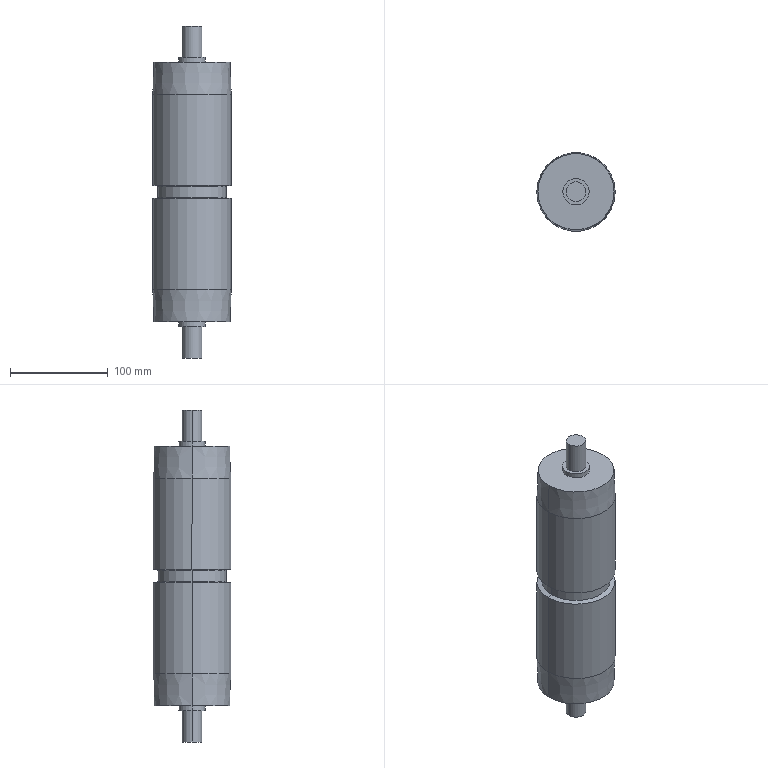Component | SolidWorks | Q1-A12-S21-Q1C.SLDASQ-1_Q1-A12-S21-Q1C-02A-1 | 1 solid | 28 faces | box 80 x 80 x 339.1 mm | volume 1333464 mm3 | cylinder 14 | cone 8 | plane 6 | commonest cylinder face diameters 27 x4 20 x4 80 x4 70 x2 | material SUJ2
build123d program:
from build123d import *


with BuildPart() as part:
    # Sketch1 → Revolve1 (revolve)
    with BuildSketch(Plane.XY, mode=Mode.PRIVATE) as revolve1_sk:
        Polygon((-132.5, 40), (132.5, 40), (132.5, 13.5), (137.45, 13.5), (137.45, 10), (169.55, 10), (169.55, 0), (-169.55, 0), (-169.55, 10), (-137.45, 10), (-137.45, 13.5), (-132.5, 13.5), align=None)
    revolve(revolve1_sk.sketch.rotate(Axis((-250, 0, 0), (1, 0, 0)), 180), axis=Axis((-250, 0, 0), (1, 0, 0)))

    # Sketch4 → Cut-Revolve1 (revolve, cut)
    with BuildSketch(Plane.XY):
        Polygon((-7, 40), (-5.9, 35), (5.9, 35), (7, 40), align=None)
    revolve(axis=Axis((-250, 0, 0), (-1, 0, 0)), mode=Mode.SUBTRACT)

    # Sketch5 → Cut-Revolve2 (revolve, cut)
    with BuildSketch(Plane.XY):
        Polygon((-132.5, 38.865), (-100, 40), (-132.5, 40), align=None)
        Polygon((132.5, 40), (100, 40), (132.5, 38.865), align=None)
    revolve(axis=Axis((-250, 0, 0), (-1, 0, 0)), mode=Mode.SUBTRACT)


solid = part.part

# Placed as in the assembly
solid = solid.moved(Location((2148, 0, 0), (0, 90, 0)))
STEP:
#1=COLOUR_RGB('',0.7922,0.8196,0.9333);
#2=FILL_AREA_STYLE_COLOUR('',#1);
#3=FILL_AREA_STYLE('',(#2));
#4=SURFACE_STYLE_FILL_AREA(#3);
#5=SURFACE_SIDE_STYLE('',(#4));
#6=SURFACE_STYLE_USAGE(.BOTH.,#5);
#7=PRESENTATION_STYLE_ASSIGNMENT((#6));
#8=CARTESIAN_POINT('',(84.035,0.,5.411));
#9=VERTEX_POINT('',#8);
#10=CARTESIAN_POINT('',(85.098,0.,5.411));
#11=VERTEX_POINT('',#10);
#12=CARTESIAN_POINT('',(84.567,0.,5.411));
#13=DIRECTION('',(-0.,-0.,-1.));
#14=DIRECTION('',(-1.,0.,0.));
#15=AXIS2_PLACEMENT_3D('',#12,#13,#14);
#16=CIRCLE('',#15,0.5315);
#17=EDGE_CURVE('',#9,#11,#16,.T.);
#18=ORIENTED_EDGE('',*,*,#17,.T.);
#19=CARTESIAN_POINT('',(85.098,0.,5.217));
#20=VERTEX_POINT('',#19);
#21=CARTESIAN_POINT('',(85.098,0.,-9.843));
#22=DIRECTION('',(-0.,-0.,-1.));
#23=VECTOR('',#22,39.37);
#24=LINE('',#21,#23);
#25=EDGE_CURVE('',#11,#20,#24,.T.);
#26=ORIENTED_EDGE('',*,*,#25,.T.);
#27=CARTESIAN_POINT('',(84.035,0.,5.217));
#28=VERTEX_POINT('',#27);
#29=CARTESIAN_POINT('',(84.567,0.,5.217));
#30=DIRECTION('',(-0.,-0.,-1.));
#31=DIRECTION('',(-1.,0.,0.));
#32=AXIS2_PLACEMENT_3D('',#29,#30,#31);
#33=CIRCLE('',#32,0.5315);
#34=EDGE_CURVE('',#28,#20,#33,.T.);
#35=ORIENTED_EDGE('',*,*,#34,.F.);
#36=CARTESIAN_POINT('',(84.035,0.,-9.843));
#37=DIRECTION('',(-0.,-0.,-1.));
#38=VECTOR('',#37,39.37);
#39=LINE('',#36,#38);
#40=EDGE_CURVE('',#9,#28,#39,.T.);
#41=ORIENTED_EDGE('',*,*,#40,.F.);
#42=EDGE_LOOP('',(#18,#26,#35,#41));
#43=FACE_OUTER_BOUND('',#42,.T.);
#44=CARTESIAN_POINT('',(84.567,0.,-9.843));
#45=DIRECTION('',(-0.,-0.,-1.));
#46=DIRECTION('',(-1.,0.,0.));
#47=AXIS2_PLACEMENT_3D('',#44,#45,#46);
#48=CYLINDRICAL_SURFACE('',#47,0.5315);
#49=ADVANCED_FACE('',(#43),#48,.T.);
#50=CARTESIAN_POINT('',(84.173,0.,6.675));
#51=VERTEX_POINT('',#50);
#52=CARTESIAN_POINT('',(84.961,0.,6.675));
#53=VERTEX_POINT('',#52);
#54=CARTESIAN_POINT('',(84.567,0.,6.675));
#55=DIRECTION('',(-0.,-0.,-1.));
#56=DIRECTION('',(-1.,0.,0.));
#57=AXIS2_PLACEMENT_3D('',#54,#55,#56);
#58=CIRCLE('',#57,0.3937);
#59=EDGE_CURVE('',#51,#53,#58,.T.);
#60=ORIENTED_EDGE('',*,*,#59,.T.);
#61=CARTESIAN_POINT('',(84.961,0.,5.411));
#62=VERTEX_POINT('',#61);
#63=CARTESIAN_POINT('',(84.961,0.,-9.843));
#64=DIRECTION('',(-0.,-0.,-1.));
#65=VECTOR('',#64,39.37);
#66=LINE('',#63,#65);
#67=EDGE_CURVE('',#53,#62,#66,.T.);
#68=ORIENTED_EDGE('',*,*,#67,.T.);
#69=CARTESIAN_POINT('',(84.173,0.,5.411));
#70=VERTEX_POINT('',#69);
#71=CARTESIAN_POINT('',(84.567,0.,5.411));
#72=DIRECTION('',(-0.,-0.,-1.));
#73=DIRECTION('',(-1.,0.,0.));
#74=AXIS2_PLACEMENT_3D('',#71,#72,#73);
#75=CIRCLE('',#74,0.3937);
#76=EDGE_CURVE('',#70,#62,#75,.T.);
#77=ORIENTED_EDGE('',*,*,#76,.F.);
#78=CARTESIAN_POINT('',(84.173,0.,-9.843));
#79=DIRECTION('',(-0.,-0.,-1.));
#80=VECTOR('',#79,39.37);
#81=LINE('',#78,#80);
#82=EDGE_CURVE('',#51,#70,#81,.T.);
#83=ORIENTED_EDGE('',*,*,#82,.F.);
#84=EDGE_LOOP('',(#60,#68,#77,#83));
#85=FACE_OUTER_BOUND('',#84,.T.);
#86=CARTESIAN_POINT('',(84.567,0.,-9.843));
#87=DIRECTION('',(-0.,-0.,-1.));
#88=DIRECTION('',(-1.,0.,0.));
#89=AXIS2_PLACEMENT_3D('',#86,#87,#88);
#90=CYLINDRICAL_SURFACE('',#89,0.3937);
#91=ADVANCED_FACE('',(#85),#90,.T.);
#92=CARTESIAN_POINT('',(86.097,0.,5.217));
#93=VERTEX_POINT('',#92);
#94=CARTESIAN_POINT('',(83.037,0.,5.217));
#95=VERTEX_POINT('',#94);
#96=CARTESIAN_POINT('',(84.567,0.,5.217));
#97=DIRECTION('',(0.,0.,1.));
#98=DIRECTION('',(1.,-0.,0.));
#99=AXIS2_PLACEMENT_3D('',#96,#97,#98);
#100=CIRCLE('',#99,1.53);
#101=EDGE_CURVE('',#93,#95,#100,.T.);
#102=ORIENTED_EDGE('',*,*,#101,.F.);
#103=CARTESIAN_POINT('',(86.142,0.,3.937));
#104=VERTEX_POINT('',#103);
#105=CARTESIAN_POINT('',(86.142,0.,3.937));
#106=DIRECTION('',(0.0349,-0.,-0.9994));
#107=VECTOR('',#106,39.37);
#108=LINE('',#105,#107);
#109=EDGE_CURVE('',#93,#104,#108,.T.);
#110=ORIENTED_EDGE('',*,*,#109,.T.);
#111=CARTESIAN_POINT('',(82.992,0.,3.937));
#112=VERTEX_POINT('',#111);
#113=CARTESIAN_POINT('',(84.567,0.,3.937));
#114=DIRECTION('',(0.,0.,1.));
#115=DIRECTION('',(1.,-0.,0.));
#116=AXIS2_PLACEMENT_3D('',#113,#114,#115);
#117=CIRCLE('',#116,1.575);
#118=EDGE_CURVE('',#104,#112,#117,.T.);
#119=ORIENTED_EDGE('',*,*,#118,.T.);
#120=CARTESIAN_POINT('',(82.992,0.,3.937));
#121=DIRECTION('',(-0.0349,-0.,-0.9994));
#122=VECTOR('',#121,39.37);
#123=LINE('',#120,#122);
#124=EDGE_CURVE('',#95,#112,#123,.T.);
#125=ORIENTED_EDGE('',*,*,#124,.F.);
#126=EDGE_LOOP('',(#102,#110,#119,#125));
#127=FACE_OUTER_BOUND('',#126,.T.);
#128=CARTESIAN_POINT('',(84.567,0.,3.937));
#129=DIRECTION('',(-0.,-0.,-1.));
#130=DIRECTION('',(-1.,0.,0.));
#131=AXIS2_PLACEMENT_3D('',#128,#129,#130);
#132=CONICAL_SURFACE('',#131,1.575,0.03491);
#133=ADVANCED_FACE('',(#127),#132,.T.);
#134=CARTESIAN_POINT('',(84.035,0.,-5.217));
#135=VERTEX_POINT('',#134);
#136=CARTESIAN_POINT('',(85.098,0.,-5.217));
#137=VERTEX_POINT('',#136);
#138=CARTESIAN_POINT('',(84.567,0.,-5.217));
#139=DIRECTION('',(-0.,-0.,-1.));
#140=DIRECTION('',(-1.,0.,0.));
#141=AXIS2_PLACEMENT_3D('',#138,#139,#140);
#142=CIRCLE('',#141,0.5315);
#143=EDGE_CURVE('',#135,#137,#142,.T.);
#144=ORIENTED_EDGE('',*,*,#143,.T.);
#145=CARTESIAN_POINT('',(85.098,0.,-5.411));
#146=VERTEX_POINT('',#145);
#147=CARTESIAN_POINT('',(85.098,0.,-9.843));
#148=DIRECTION('',(-0.,-0.,-1.));
#149=VECTOR('',#148,39.37);
#150=LINE('',#147,#149);
#151=EDGE_CURVE('',#137,#146,#150,.T.);
#152=ORIENTED_EDGE('',*,*,#151,.T.);
#153=CARTESIAN_POINT('',(84.035,0.,-5.411));
#154=VERTEX_POINT('',#153);
#155=CARTESIAN_POINT('',(84.567,0.,-5.411));
#156=DIRECTION('',(-0.,-0.,-1.));
#157=DIRECTION('',(-1.,0.,0.));
#158=AXIS2_PLACEMENT_3D('',#155,#156,#157);
#159=CIRCLE('',#158,0.5315);
#160=EDGE_CURVE('',#154,#146,#159,.T.);
#161=ORIENTED_EDGE('',*,*,#160,.F.);
#162=CARTESIAN_POINT('',(84.035,0.,-9.843));
#163=DIRECTION('',(-0.,-0.,-1.));
#164=VECTOR('',#163,39.37);
#165=LINE('',#162,#164);
#166=EDGE_CURVE('',#135,#154,#165,.T.);
#167=ORIENTED_EDGE('',*,*,#166,.F.);
#168=EDGE_LOOP('',(#144,#152,#161,#167));
#169=FACE_OUTER_BOUND('',#168,.T.);
#170=CARTESIAN_POINT('',(84.567,0.,-9.843));
#171=DIRECTION('',(-0.,-0.,-1.));
#172=DIRECTION('',(-1.,0.,0.));
#173=AXIS2_PLACEMENT_3D('',#170,#171,#172);
#174=CYLINDRICAL_SURFACE('',#173,0.5315);
#175=ADVANCED_FACE('',(#169),#174,.T.);
#176=CARTESIAN_POINT('',(84.173,0.,-5.411));
#177=VERTEX_POINT('',#176);
#178=CARTESIAN_POINT('',(84.961,0.,-5.411));
#179=VERTEX_POINT('',#178);
#180=CARTESIAN_POINT('',(84.567,0.,-5.411));
#181=DIRECTION('',(-0.,-0.,-1.));
#182=DIRECTION('',(-1.,0.,0.));
#183=AXIS2_PLACEMENT_3D('',#180,#181,#182);
#184=CIRCLE('',#183,0.3937);
#185=EDGE_CURVE('',#177,#179,#184,.T.);
#186=ORIENTED_EDGE('',*,*,#185,.T.);
#187=CARTESIAN_POINT('',(84.961,0.,-6.675));
#188=VERTEX_POINT('',#187);
#189=CARTESIAN_POINT('',(84.961,0.,-9.843));
#190=DIRECTION('',(-0.,-0.,-1.));
#191=VECTOR('',#190,39.37);
#192=LINE('',#189,#191);
#193=EDGE_CURVE('',#179,#188,#192,.T.);
#194=ORIENTED_EDGE('',*,*,#193,.T.);
#195=CARTESIAN_POINT('',(84.173,0.,-6.675));
#196=VERTEX_POINT('',#195);
#197=CARTESIAN_POINT('',(84.567,0.,-6.675));
#198=DIRECTION('',(-0.,-0.,-1.));
#199=DIRECTION('',(-1.,0.,0.));
#200=AXIS2_PLACEMENT_3D('',#197,#198,#199);
#201=CIRCLE('',#200,0.3937);
#202=EDGE_CURVE('',#196,#188,#201,.T.);
#203=ORIENTED_EDGE('',*,*,#202,.F.);
#204=CARTESIAN_POINT('',(84.173,0.,-9.843));
#205=DIRECTION('',(-0.,-0.,-1.));
#206=VECTOR('',#205,39.37);
#207=LINE('',#204,#206);
#208=EDGE_CURVE('',#177,#196,#207,.T.);
#209=ORIENTED_EDGE('',*,*,#208,.F.);
#210=EDGE_LOOP('',(#186,#194,#203,#209));
#211=FACE_OUTER_BOUND('',#210,.T.);
#212=CARTESIAN_POINT('',(84.567,0.,-9.843));
#213=DIRECTION('',(-0.,-0.,-1.));
#214=DIRECTION('',(-1.,0.,0.));
#215=AXIS2_PLACEMENT_3D('',#212,#213,#214);
#216=CYLINDRICAL_SURFACE('',#215,0.3937);
#217=ADVANCED_FACE('',(#211),#216,.T.);
#218=CARTESIAN_POINT('',(86.097,0.,-5.217));
#219=VERTEX_POINT('',#218);
#220=CARTESIAN_POINT('',(83.037,0.,-5.217));
#221=VERTEX_POINT('',#220);
#222=CARTESIAN_POINT('',(84.567,0.,-5.217));
#223=DIRECTION('',(0.,0.,1.));
#224=DIRECTION('',(1.,-0.,0.));
#225=AXIS2_PLACEMENT_3D('',#222,#223,#224);
#226=CIRCLE('',#225,1.53);
#227=EDGE_CURVE('',#219,#221,#226,.T.);
#228=ORIENTED_EDGE('',*,*,#227,.T.);
#229=CARTESIAN_POINT('',(82.992,0.,-3.937));
#230=VERTEX_POINT('',#229);
#231=CARTESIAN_POINT('',(83.037,0.,-5.217));
#232=DIRECTION('',(-0.0349,0.,0.9994));
#233=VECTOR('',#232,39.37);
#234=LINE('',#231,#233);
#235=EDGE_CURVE('',#221,#230,#234,.T.);
#236=ORIENTED_EDGE('',*,*,#235,.T.);
#237=CARTESIAN_POINT('',(86.142,0.,-3.937));
#238=VERTEX_POINT('',#237);
#239=CARTESIAN_POINT('',(84.567,0.,-3.937));
#240=DIRECTION('',(0.,0.,1.));
#241=DIRECTION('',(1.,-0.,0.));
#242=AXIS2_PLACEMENT_3D('',#239,#240,#241);
#243=CIRCLE('',#242,1.575);
#244=EDGE_CURVE('',#238,#230,#243,.T.);
#245=ORIENTED_EDGE('',*,*,#244,.F.);
#246=CARTESIAN_POINT('',(86.097,0.,-5.217));
#247=DIRECTION('',(0.0349,0.,0.9994));
#248=VECTOR('',#247,39.37);
#249=LINE('',#246,#248);
#250=EDGE_CURVE('',#219,#238,#249,.T.);
#251=ORIENTED_EDGE('',*,*,#250,.F.);
#252=EDGE_LOOP('',(#228,#236,#245,#251));
#253=FACE_OUTER_BOUND('',#252,.T.);
#254=CARTESIAN_POINT('',(84.567,0.,-5.217));
#255=DIRECTION('',(0.,0.,1.));
#256=DIRECTION('',(1.,-0.,0.));
#257=AXIS2_PLACEMENT_3D('',#254,#255,#256);
#258=CONICAL_SURFACE('',#257,1.53,0.03491);
#259=ADVANCED_FACE('',(#253),#258,.T.);
#260=ORIENTED_EDGE('',*,*,#118,.F.);
#261=CARTESIAN_POINT('',(86.142,0.,0.2756));
#262=VERTEX_POINT('',#261);
#263=CARTESIAN_POINT('',(86.142,0.,-9.843));
#264=DIRECTION('',(-0.,-0.,-1.));
#265=VECTOR('',#264,39.37);
#266=LINE('',#263,#265);
#267=EDGE_CURVE('',#104,#262,#266,.T.);
#268=ORIENTED_EDGE('',*,*,#267,.T.);
#269=CARTESIAN_POINT('',(82.992,0.,0.2756));
#270=VERTEX_POINT('',#269);
#271=CARTESIAN_POINT('',(84.567,0.,0.2756));
#272=DIRECTION('',(0.,0.,1.));
#273=DIRECTION('',(1.,-0.,-0.));
#274=AXIS2_PLACEMENT_3D('',#271,#272,#273);
#275=CIRCLE('',#274,1.575);
#276=EDGE_CURVE('',#262,#270,#275,.T.);
#277=ORIENTED_EDGE('',*,*,#276,.T.);
#278=CARTESIAN_POINT('',(82.992,0.,-9.843));
#279=DIRECTION('',(-0.,-0.,-1.));
#280=VECTOR('',#279,39.37);
#281=LINE('',#278,#280);
#282=EDGE_CURVE('',#112,#270,#281,.T.);
#283=ORIENTED_EDGE('',*,*,#282,.F.);
#284=EDGE_LOOP('',(#260,#268,#277,#283));
#285=FACE_OUTER_BOUND('',#284,.T.);
#286=CARTESIAN_POINT('',(84.567,0.,-9.843));
#287=DIRECTION('',(-0.,-0.,-1.));
#288=DIRECTION('',(-1.,0.,0.));
#289=AXIS2_PLACEMENT_3D('',#286,#287,#288);
#290=CYLINDRICAL_SURFACE('',#289,1.575);
#291=ADVANCED_FACE('',(#285),#290,.T.);
#292=CARTESIAN_POINT('',(85.945,0.,0.2323));
#293=VERTEX_POINT('',#292);
#294=CARTESIAN_POINT('',(83.189,0.,0.2323));
#295=VERTEX_POINT('',#294);
#296=CARTESIAN_POINT('',(84.567,0.,0.2323));
#297=DIRECTION('',(0.,0.,1.));
#298=DIRECTION('',(1.,-0.,-0.));
#299=AXIS2_PLACEMENT_3D('',#296,#297,#298);
#300=CIRCLE('',#299,1.378);
#301=EDGE_CURVE('',#293,#295,#300,.T.);
#302=ORIENTED_EDGE('',*,*,#301,.T.);
#303=CARTESIAN_POINT('',(83.189,0.,0.2323));
#304=DIRECTION('',(-0.9766,0.,0.2149));
#305=VECTOR('',#304,39.37);
#306=LINE('',#303,#305);
#307=EDGE_CURVE('',#295,#270,#306,.T.);
#308=ORIENTED_EDGE('',*,*,#307,.T.);
#309=ORIENTED_EDGE('',*,*,#276,.F.);
#310=CARTESIAN_POINT('',(85.945,0.,0.2323));
#311=DIRECTION('',(0.9766,-0.,0.2149));
#312=VECTOR('',#311,39.37);
#313=LINE('',#310,#312);
#314=EDGE_CURVE('',#293,#262,#313,.T.);
#315=ORIENTED_EDGE('',*,*,#314,.F.);
#316=EDGE_LOOP('',(#302,#308,#309,#315));
#317=FACE_OUTER_BOUND('',#316,.T.);
#318=CARTESIAN_POINT('',(84.567,0.,0.2323));
#319=DIRECTION('',(0.,0.,1.));
#320=DIRECTION('',(1.,-0.,-0.));
#321=AXIS2_PLACEMENT_3D('',#318,#319,#320);
#322=CONICAL_SURFACE('',#321,1.378,1.354);
#323=ADVANCED_FACE('',(#317),#322,.T.);
#324=CARTESIAN_POINT('',(85.945,0.,-0.2323));
#325=VERTEX_POINT('',#324);
#326=CARTESIAN_POINT('',(83.189,0.,-0.2323));
#327=VERTEX_POINT('',#326);
#328=CARTESIAN_POINT('',(84.567,0.,-0.2323));
#329=DIRECTION('',(0.,0.,1.));
#330=DIRECTION('',(1.,-0.,-0.));
#331=AXIS2_PLACEMENT_3D('',#328,#329,#330);
#332=CIRCLE('',#331,1.378);
#333=EDGE_CURVE('',#325,#327,#332,.T.);
#334=ORIENTED_EDGE('',*,*,#333,.T.);
#335=CARTESIAN_POINT('',(83.189,0.,5.217));
#336=DIRECTION('',(0.,0.,1.));
#337=VECTOR('',#336,39.37);
#338=LINE('',#335,#337);
#339=EDGE_CURVE('',#327,#295,#338,.T.);
#340=ORIENTED_EDGE('',*,*,#339,.T.);
#341=ORIENTED_EDGE('',*,*,#301,.F.);
#342=CARTESIAN_POINT('',(85.945,0.,5.217));
#343=DIRECTION('',(0.,0.,1.));
#344=VECTOR('',#343,39.37);
#345=LINE('',#342,#344);
#346=EDGE_CURVE('',#325,#293,#345,.T.);
#347=ORIENTED_EDGE('',*,*,#346,.F.);
#348=EDGE_LOOP('',(#334,#340,#341,#347));
#349=FACE_OUTER_BOUND('',#348,.T.);
#350=CARTESIAN_POINT('',(84.567,0.,5.217));
#351=DIRECTION('',(0.,0.,1.));
#352=DIRECTION('',(1.,-0.,0.));
#353=AXIS2_PLACEMENT_3D('',#350,#351,#352);
#354=CYLINDRICAL_SURFACE('',#353,1.378);
#355=ADVANCED_FACE('',(#349),#354,.T.);
#356=ORIENTED_EDGE('',*,*,#333,.F.);
#357=CARTESIAN_POINT('',(86.142,0.,-0.2756));
#358=VERTEX_POINT('',#357);
#359=CARTESIAN_POINT('',(86.142,0.,-0.2756));
#360=DIRECTION('',(0.9766,0.,-0.2149));
#361=VECTOR('',#360,39.37);
#362=LINE('',#359,#361);
#363=EDGE_CURVE('',#325,#358,#362,.T.);
#364=ORIENTED_EDGE('',*,*,#363,.T.);
#365=CARTESIAN_POINT('',(82.992,0.,-0.2756));
#366=VERTEX_POINT('',#365);
#367=CARTESIAN_POINT('',(84.567,0.,-0.2756));
#368=DIRECTION('',(0.,0.,1.));
#369=DIRECTION('',(1.,-0.,-0.));
#370=AXIS2_PLACEMENT_3D('',#367,#368,#369);
#371=CIRCLE('',#370,1.575);
#372=EDGE_CURVE('',#358,#366,#371,.T.);
#373=ORIENTED_EDGE('',*,*,#372,.T.);
#374=CARTESIAN_POINT('',(82.992,0.,-0.2756));
#375=DIRECTION('',(-0.9766,0.,-0.2149));
#376=VECTOR('',#375,39.37);
#377=LINE('',#374,#376);
#378=EDGE_CURVE('',#327,#366,#377,.T.);
#379=ORIENTED_EDGE('',*,*,#378,.F.);
#380=EDGE_LOOP('',(#356,#364,#373,#379));
#381=FACE_OUTER_BOUND('',#380,.T.);
#382=CARTESIAN_POINT('',(84.567,0.,-0.2756));
#383=DIRECTION('',(-0.,-0.,-1.));
#384=DIRECTION('',(-1.,0.,0.));
#385=AXIS2_PLACEMENT_3D('',#382,#383,#384);
#386=CONICAL_SURFACE('',#385,1.575,1.354);
#387=ADVANCED_FACE('',(#381),#386,.T.);
#388=ORIENTED_EDGE('',*,*,#372,.F.);
#389=CARTESIAN_POINT('',(86.142,0.,-9.843));
#390=DIRECTION('',(-0.,-0.,-1.));
#391=VECTOR('',#390,39.37);
#392=LINE('',#389,#391);
#393=EDGE_CURVE('',#358,#238,#392,.T.);
#394=ORIENTED_EDGE('',*,*,#393,.T.);
#395=ORIENTED_EDGE('',*,*,#244,.T.);
#396=CARTESIAN_POINT('',(82.992,0.,-9.843));
#397=DIRECTION('',(-0.,-0.,-1.));
#398=VECTOR('',#397,39.37);
#399=LINE('',#396,#398);
#400=EDGE_CURVE('',#366,#230,#399,.T.);
#401=ORIENTED_EDGE('',*,*,#400,.F.);
#402=EDGE_LOOP('',(#388,#394,#395,#401));
#403=FACE_OUTER_BOUND('',#402,.T.);
#404=CARTESIAN_POINT('',(84.567,0.,-9.843));
#405=DIRECTION('',(-0.,-0.,-1.));
#406=DIRECTION('',(-1.,0.,0.));
#407=AXIS2_PLACEMENT_3D('',#404,#405,#406);
#408=CYLINDRICAL_SURFACE('',#407,1.575);
#409=ADVANCED_FACE('',(#403),#408,.T.);
#410=ORIENTED_EDGE('',*,*,#393,.F.);
#411=CARTESIAN_POINT('',(84.567,0.,-0.2756));
#412=DIRECTION('',(0.,0.,1.));
#413=DIRECTION('',(1.,-0.,-0.));
#414=AXIS2_PLACEMENT_3D('',#411,#412,#413);
#415=CIRCLE('',#414,1.575);
#416=EDGE_CURVE('',#366,#358,#415,.T.);
#417=ORIENTED_EDGE('',*,*,#416,.F.);
#418=ORIENTED_EDGE('',*,*,#400,.T.);
#419=CARTESIAN_POINT('',(84.567,0.,-3.937));
#420=DIRECTION('',(0.,0.,1.));
#421=DIRECTION('',(1.,-0.,0.));
#422=AXIS2_PLACEMENT_3D('',#419,#420,#421);
#423=CIRCLE('',#422,1.575);
#424=EDGE_CURVE('',#230,#238,#423,.T.);
#425=ORIENTED_EDGE('',*,*,#424,.T.);
#426=EDGE_LOOP('',(#410,#417,#418,#425));
#427=FACE_OUTER_BOUND('',#426,.T.);
#428=CARTESIAN_POINT('',(84.567,0.,-9.843));
#429=DIRECTION('',(-0.,-0.,-1.));
#430=DIRECTION('',(-1.,0.,0.));
#431=AXIS2_PLACEMENT_3D('',#428,#429,#430);
#432=CYLINDRICAL_SURFACE('',#431,1.575);
#433=ADVANCED_FACE('',(#427),#432,.T.);
#434=ORIENTED_EDGE('',*,*,#363,.F.);
#435=CARTESIAN_POINT('',(84.567,0.,-0.2323));
#436=DIRECTION('',(0.,0.,1.));
#437=DIRECTION('',(1.,-0.,-0.));
#438=AXIS2_PLACEMENT_3D('',#435,#436,#437);
#439=CIRCLE('',#438,1.378);
#440=EDGE_CURVE('',#327,#325,#439,.T.);
#441=ORIENTED_EDGE('',*,*,#440,.F.);
#442=ORIENTED_EDGE('',*,*,#378,.T.);
#443=ORIENTED_EDGE('',*,*,#416,.T.);
#444=EDGE_LOOP('',(#434,#441,#442,#443));
#445=FACE_OUTER_BOUND('',#444,.T.);
#446=CARTESIAN_POINT('',(84.567,0.,-0.2756));
#447=DIRECTION('',(-0.,-0.,-1.));
#448=DIRECTION('',(-1.,0.,0.));
#449=AXIS2_PLACEMENT_3D('',#446,#447,#448);
#450=CONICAL_SURFACE('',#449,1.575,1.354);
#451=ADVANCED_FACE('',(#445),#450,.T.);
#452=ORIENTED_EDGE('',*,*,#339,.F.);
#453=ORIENTED_EDGE('',*,*,#440,.T.);
#454=ORIENTED_EDGE('',*,*,#346,.T.);
#455=CARTESIAN_POINT('',(84.567,0.,0.2323));
#456=DIRECTION('',(0.,0.,1.));
#457=DIRECTION('',(1.,-0.,-0.));
#458=AXIS2_PLACEMENT_3D('',#455,#456,#457);
#459=CIRCLE('',#458,1.378);
#460=EDGE_CURVE('',#295,#293,#459,.T.);
#461=ORIENTED_EDGE('',*,*,#460,.F.);
#462=EDGE_LOOP('',(#452,#453,#454,#461));
#463=FACE_OUTER_BOUND('',#462,.T.);
#464=CARTESIAN_POINT('',(84.567,0.,5.217));
#465=DIRECTION('',(0.,0.,1.));
#466=DIRECTION('',(1.,-0.,0.));
#467=AXIS2_PLACEMENT_3D('',#464,#465,#466);
#468=CYLINDRICAL_SURFACE('',#467,1.378);
#469=ADVANCED_FACE('',(#463),#468,.T.);
#470=ORIENTED_EDGE('',*,*,#307,.F.);
#471=ORIENTED_EDGE('',*,*,#460,.T.);
#472=ORIENTED_EDGE('',*,*,#314,.T.);
#473=CARTESIAN_POINT('',(84.567,0.,0.2756));
#474=DIRECTION('',(0.,0.,1.));
#475=DIRECTION('',(1.,-0.,-0.));
#476=AXIS2_PLACEMENT_3D('',#473,#474,#475);
#477=CIRCLE('',#476,1.575);
#478=EDGE_CURVE('',#270,#262,#477,.T.);
#479=ORIENTED_EDGE('',*,*,#478,.F.);
#480=EDGE_LOOP('',(#470,#471,#472,#479));
#481=FACE_OUTER_BOUND('',#480,.T.);
#482=CARTESIAN_POINT('',(84.567,0.,0.2323));
#483=DIRECTION('',(0.,0.,1.));
#484=DIRECTION('',(1.,-0.,-0.));
#485=AXIS2_PLACEMENT_3D('',#482,#483,#484);
#486=CONICAL_SURFACE('',#485,1.378,1.354);
#487=ADVANCED_FACE('',(#481),#486,.T.);
#488=ORIENTED_EDGE('',*,*,#267,.F.);
#489=CARTESIAN_POINT('',(84.567,0.,3.937));
#490=DIRECTION('',(0.,0.,1.));
#491=DIRECTION('',(1.,-0.,0.));
#492=AXIS2_PLACEMENT_3D('',#489,#490,#491);
#493=CIRCLE('',#492,1.575);
#494=EDGE_CURVE('',#112,#104,#493,.T.);
#495=ORIENTED_EDGE('',*,*,#494,.F.);
#496=ORIENTED_EDGE('',*,*,#282,.T.);
#497=ORIENTED_EDGE('',*,*,#478,.T.);
#498=EDGE_LOOP('',(#488,#495,#496,#497));
#499=FACE_OUTER_BOUND('',#498,.T.);
#500=CARTESIAN_POINT('',(84.567,0.,-9.843));
#501=DIRECTION('',(-0.,-0.,-1.));
#502=DIRECTION('',(-1.,0.,0.));
#503=AXIS2_PLACEMENT_3D('',#500,#501,#502);
#504=CYLINDRICAL_SURFACE('',#503,1.575);
#505=ADVANCED_FACE('',(#499),#504,.T.);
#506=ORIENTED_EDGE('',*,*,#235,.F.);
#507=CARTESIAN_POINT('',(84.567,0.,-5.217));
#508=DIRECTION('',(0.,0.,1.));
#509=DIRECTION('',(1.,-0.,0.));
#510=AXIS2_PLACEMENT_3D('',#507,#508,#509);
#511=CIRCLE('',#510,1.53);
#512=EDGE_CURVE('',#221,#219,#511,.T.);
#513=ORIENTED_EDGE('',*,*,#512,.T.);
#514=ORIENTED_EDGE('',*,*,#250,.T.);
#515=ORIENTED_EDGE('',*,*,#424,.F.);
#516=EDGE_LOOP('',(#506,#513,#514,#515));
#517=FACE_OUTER_BOUND('',#516,.T.);
#518=CARTESIAN_POINT('',(84.567,0.,-5.217));
#519=DIRECTION('',(0.,0.,1.));
#520=DIRECTION('',(1.,-0.,0.));
#521=AXIS2_PLACEMENT_3D('',#518,#519,#520);
#522=CONICAL_SURFACE('',#521,1.53,0.03491);
#523=ADVANCED_FACE('',(#517),#522,.T.);
#524=ORIENTED_EDGE('',*,*,#202,.T.);
#525=CARTESIAN_POINT('',(84.567,0.,-6.675));
#526=DIRECTION('',(-0.,-0.,-1.));
#527=DIRECTION('',(-1.,0.,0.));
#528=AXIS2_PLACEMENT_3D('',#525,#526,#527);
#529=CIRCLE('',#528,0.3937);
#530=EDGE_CURVE('',#188,#196,#529,.T.);
#531=ORIENTED_EDGE('',*,*,#530,.T.);
#532=EDGE_LOOP('',(#524,#531));
#533=FACE_OUTER_BOUND('',#532,.T.);
#534=CARTESIAN_POINT('',(84.961,0.,-6.675));
#535=DIRECTION('',(0.,0.,1.));
#536=DIRECTION('',(1.,-0.,-0.));
#537=AXIS2_PLACEMENT_3D('',#534,#535,#536);
#538=PLANE('',#537);
#539=ADVANCED_FACE('',(#533),#538,.F.);
#540=ORIENTED_EDGE('',*,*,#193,.F.);
#541=CARTESIAN_POINT('',(84.567,0.,-5.411));
#542=DIRECTION('',(-0.,-0.,-1.));
#543=DIRECTION('',(-1.,0.,0.));
#544=AXIS2_PLACEMENT_3D('',#541,#542,#543);
#545=CIRCLE('',#544,0.3937);
#546=EDGE_CURVE('',#179,#177,#545,.T.);
#547=ORIENTED_EDGE('',*,*,#546,.T.);
#548=ORIENTED_EDGE('',*,*,#208,.T.);
#549=ORIENTED_EDGE('',*,*,#530,.F.);
#550=EDGE_LOOP('',(#540,#547,#548,#549));
#551=FACE_OUTER_BOUND('',#550,.T.);
#552=CARTESIAN_POINT('',(84.567,0.,-9.843));
#553=DIRECTION('',(-0.,-0.,-1.));
#554=DIRECTION('',(-1.,0.,0.));
#555=AXIS2_PLACEMENT_3D('',#552,#553,#554);
#556=CYLINDRICAL_SURFACE('',#555,0.3937);
#557=ADVANCED_FACE('',(#551),#556,.T.);
#558=ORIENTED_EDGE('',*,*,#185,.F.);
#559=ORIENTED_EDGE('',*,*,#546,.F.);
#560=EDGE_LOOP('',(#558,#559));
#561=FACE_BOUND('',#560,.T.);
#562=ORIENTED_EDGE('',*,*,#160,.T.);
#563=CARTESIAN_POINT('',(84.567,0.,-5.411));
#564=DIRECTION('',(-0.,-0.,-1.));
#565=DIRECTION('',(-1.,0.,0.));
#566=AXIS2_PLACEMENT_3D('',#563,#564,#565);
#567=CIRCLE('',#566,0.5315);
#568=EDGE_CURVE('',#146,#154,#567,.T.);
#569=ORIENTED_EDGE('',*,*,#568,.T.);
#570=EDGE_LOOP('',(#562,#569));
#571=FACE_OUTER_BOUND('',#570,.T.);
#572=CARTESIAN_POINT('',(85.098,0.,-5.411));
#573=DIRECTION('',(0.,0.,1.));
#574=DIRECTION('',(1.,-0.,-0.));
#575=AXIS2_PLACEMENT_3D('',#572,#573,#574);
#576=PLANE('',#575);
#577=ADVANCED_FACE('',(#561,#571),#576,.F.);
#578=ORIENTED_EDGE('',*,*,#151,.F.);
#579=CARTESIAN_POINT('',(84.567,0.,-5.217));
#580=DIRECTION('',(-0.,-0.,-1.));
#581=DIRECTION('',(-1.,0.,0.));
#582=AXIS2_PLACEMENT_3D('',#579,#580,#581);
#583=CIRCLE('',#582,0.5315);
#584=EDGE_CURVE('',#137,#135,#583,.T.);
#585=ORIENTED_EDGE('',*,*,#584,.T.);
#586=ORIENTED_EDGE('',*,*,#166,.T.);
#587=ORIENTED_EDGE('',*,*,#568,.F.);
#588=EDGE_LOOP('',(#578,#585,#586,#587));
#589=FACE_OUTER_BOUND('',#588,.T.);
#590=CARTESIAN_POINT('',(84.567,0.,-9.843));
#591=DIRECTION('',(-0.,-0.,-1.));
#592=DIRECTION('',(-1.,0.,0.));
#593=AXIS2_PLACEMENT_3D('',#590,#591,#592);
#594=CYLINDRICAL_SURFACE('',#593,0.5315);
#595=ADVANCED_FACE('',(#589),#594,.T.);
#596=ORIENTED_EDGE('',*,*,#143,.F.);
#597=ORIENTED_EDGE('',*,*,#584,.F.);
#598=EDGE_LOOP('',(#596,#597));
#599=FACE_BOUND('',#598,.T.);
#600=ORIENTED_EDGE('',*,*,#227,.F.);
#601=ORIENTED_EDGE('',*,*,#512,.F.);
#602=EDGE_LOOP('',(#600,#601));
#603=FACE_OUTER_BOUND('',#602,.T.);
#604=CARTESIAN_POINT('',(85.098,0.,-5.217));
#605=DIRECTION('',(0.,0.,1.));
#606=DIRECTION('',(1.,-0.,-0.));
#607=AXIS2_PLACEMENT_3D('',#604,#605,#606);
#608=PLANE('',#607);
#609=ADVANCED_FACE('',(#599,#603),#608,.F.);
#610=ORIENTED_EDGE('',*,*,#109,.F.);
#611=CARTESIAN_POINT('',(84.567,0.,5.217));
#612=DIRECTION('',(0.,0.,1.));
#613=DIRECTION('',(1.,-0.,0.));
#614=AXIS2_PLACEMENT_3D('',#611,#612,#613);
#615=CIRCLE('',#614,1.53);
#616=EDGE_CURVE('',#95,#93,#615,.T.);
#617=ORIENTED_EDGE('',*,*,#616,.F.);
#618=ORIENTED_EDGE('',*,*,#124,.T.);
#619=ORIENTED_EDGE('',*,*,#494,.T.);
#620=EDGE_LOOP('',(#610,#617,#618,#619));
#621=FACE_OUTER_BOUND('',#620,.T.);
#622=CARTESIAN_POINT('',(84.567,0.,3.937));
#623=DIRECTION('',(-0.,-0.,-1.));
#624=DIRECTION('',(-1.,0.,0.));
#625=AXIS2_PLACEMENT_3D('',#622,#623,#624);
#626=CONICAL_SURFACE('',#625,1.575,0.03491);
#627=ADVANCED_FACE('',(#621),#626,.T.);
#628=ORIENTED_EDGE('',*,*,#59,.F.);
#629=CARTESIAN_POINT('',(84.567,0.,6.675));
#630=DIRECTION('',(-0.,-0.,-1.));
#631=DIRECTION('',(-1.,0.,0.));
#632=AXIS2_PLACEMENT_3D('',#629,#630,#631);
#633=CIRCLE('',#632,0.3937);
#634=EDGE_CURVE('',#53,#51,#633,.T.);
#635=ORIENTED_EDGE('',*,*,#634,.F.);
#636=EDGE_LOOP('',(#628,#635));
#637=FACE_OUTER_BOUND('',#636,.T.);
#638=CARTESIAN_POINT('',(84.961,0.,6.675));
#639=DIRECTION('',(-0.,-0.,-1.));
#640=DIRECTION('',(-1.,0.,0.));
#641=AXIS2_PLACEMENT_3D('',#638,#639,#640);
#642=PLANE('',#641);
#643=ADVANCED_FACE('',(#637),#642,.F.);
#644=ORIENTED_EDGE('',*,*,#67,.F.);
#645=ORIENTED_EDGE('',*,*,#634,.T.);
#646=ORIENTED_EDGE('',*,*,#82,.T.);
#647=CARTESIAN_POINT('',(84.567,0.,5.411));
#648=DIRECTION('',(-0.,-0.,-1.));
#649=DIRECTION('',(-1.,0.,0.));
#650=AXIS2_PLACEMENT_3D('',#647,#648,#649);
#651=CIRCLE('',#650,0.3937);
#652=EDGE_CURVE('',#62,#70,#651,.T.);
#653=ORIENTED_EDGE('',*,*,#652,.F.);
#654=EDGE_LOOP('',(#644,#645,#646,#653));
#655=FACE_OUTER_BOUND('',#654,.T.);
#656=CARTESIAN_POINT('',(84.567,0.,-9.843));
#657=DIRECTION('',(-0.,-0.,-1.));
#658=DIRECTION('',(-1.,0.,0.));
#659=AXIS2_PLACEMENT_3D('',#656,#657,#658);
#660=CYLINDRICAL_SURFACE('',#659,0.3937);
#661=ADVANCED_FACE('',(#655),#660,.T.);
#662=ORIENTED_EDGE('',*,*,#17,.F.);
#663=CARTESIAN_POINT('',(84.567,0.,5.411));
#664=DIRECTION('',(-0.,-0.,-1.));
#665=DIRECTION('',(-1.,0.,0.));
#666=AXIS2_PLACEMENT_3D('',#663,#664,#665);
#667=CIRCLE('',#666,0.5315);
#668=EDGE_CURVE('',#11,#9,#667,.T.);
#669=ORIENTED_EDGE('',*,*,#668,.F.);
#670=EDGE_LOOP('',(#662,#669));
#671=FACE_OUTER_BOUND('',#670,.T.);
#672=ORIENTED_EDGE('',*,*,#76,.T.);
#673=ORIENTED_EDGE('',*,*,#652,.T.);
#674=EDGE_LOOP('',(#672,#673));
#675=FACE_BOUND('',#674,.T.);
#676=CARTESIAN_POINT('',(85.098,0.,5.411));
#677=DIRECTION('',(-0.,-0.,-1.));
#678=DIRECTION('',(-1.,0.,0.));
#679=AXIS2_PLACEMENT_3D('',#676,#677,#678);
#680=PLANE('',#679);
#681=ADVANCED_FACE('',(#671,#675),#680,.F.);
#682=ORIENTED_EDGE('',*,*,#25,.F.);
#683=ORIENTED_EDGE('',*,*,#668,.T.);
#684=ORIENTED_EDGE('',*,*,#40,.T.);
#685=CARTESIAN_POINT('',(84.567,0.,5.217));
#686=DIRECTION('',(-0.,-0.,-1.));
#687=DIRECTION('',(-1.,0.,0.));
#688=AXIS2_PLACEMENT_3D('',#685,#686,#687);
#689=CIRCLE('',#688,0.5315);
#690=EDGE_CURVE('',#20,#28,#689,.T.);
#691=ORIENTED_EDGE('',*,*,#690,.F.);
#692=EDGE_LOOP('',(#682,#683,#684,#691));
#693=FACE_OUTER_BOUND('',#692,.T.);
#694=CARTESIAN_POINT('',(84.567,0.,-9.843));
#695=DIRECTION('',(-0.,-0.,-1.));
#696=DIRECTION('',(-1.,0.,0.));
#697=AXIS2_PLACEMENT_3D('',#694,#695,#696);
#698=CYLINDRICAL_SURFACE('',#697,0.5315);
#699=ADVANCED_FACE('',(#693),#698,.T.);
#700=ORIENTED_EDGE('',*,*,#34,.T.);
#701=ORIENTED_EDGE('',*,*,#690,.T.);
#702=EDGE_LOOP('',(#700,#701));
#703=FACE_BOUND('',#702,.T.);
#704=ORIENTED_EDGE('',*,*,#616,.T.);
#705=ORIENTED_EDGE('',*,*,#101,.T.);
#706=EDGE_LOOP('',(#704,#705));
#707=FACE_OUTER_BOUND('',#706,.T.);
#708=CARTESIAN_POINT('',(86.142,0.,5.217));
#709=DIRECTION('',(-0.,-0.,-1.));
#710=DIRECTION('',(-1.,0.,0.));
#711=AXIS2_PLACEMENT_3D('',#708,#709,#710);
#712=PLANE('',#711);
#713=ADVANCED_FACE('',(#703,#707),#712,.F.);
#714=CLOSED_SHELL('',(#49,#91,#133,#175,#217,#259,#291,#323,#355,#387,#409,#433,#451,#469,#487,#505,#523,#539,#557,#577,#595,#609,#627,#643,#661,#681,#699,#713));
#715=MANIFOLD_SOLID_BREP('',#714);
#716=STYLED_ITEM('',(#7),#715);
#717=PRESENTATION_LAYER_ASSIGNMENT('','',(#716));
#718=(LENGTH_UNIT()NAMED_UNIT(*)SI_UNIT($,.METRE.));
#719=LENGTH_MEASURE_WITH_UNIT(LENGTH_MEASURE(0.0254),#718);
#720=DIMENSIONAL_EXPONENTS(1.,0.,0.,0.,0.,0.,0.);
#721=(CONVERSION_BASED_UNIT('',#719)LENGTH_UNIT()NAMED_UNIT(#720));
#722=UNCERTAINTY_MEASURE_WITH_UNIT(LENGTH_MEASURE(0.00001),#721,'','');
#723=(NAMED_UNIT(*)PLANE_ANGLE_UNIT()SI_UNIT($,.RADIAN.));
#724=(NAMED_UNIT(*)SI_UNIT($,.STERADIAN.)SOLID_ANGLE_UNIT());
#725=(GEOMETRIC_REPRESENTATION_CONTEXT(3)GLOBAL_UNCERTAINTY_ASSIGNED_CONTEXT((#722))GLOBAL_UNIT_ASSIGNED_CONTEXT((#721,#723,#724))REPRESENTATION_CONTEXT('',''));
#726=MECHANICAL_DESIGN_GEOMETRIC_PRESENTATION_REPRESENTATION('',(#716),#725);
#727=CARTESIAN_POINT('',(0.,0.,0.));
#728=DIRECTION('',(0.,0.,1.));
#729=DIRECTION('',(1.,0.,0.));
#730=AXIS2_PLACEMENT_3D('',#727,#728,#729);
#731=(LENGTH_UNIT()NAMED_UNIT(*)SI_UNIT($,.METRE.));
#732=LENGTH_MEASURE_WITH_UNIT(LENGTH_MEASURE(0.0254),#731);
#733=DIMENSIONAL_EXPONENTS(1.,0.,0.,0.,0.,0.,0.);
#734=(CONVERSION_BASED_UNIT('',#732)LENGTH_UNIT()NAMED_UNIT(#733));
#735=UNCERTAINTY_MEASURE_WITH_UNIT(LENGTH_MEASURE(0.00001),#734,'','');
#736=(NAMED_UNIT(*)PLANE_ANGLE_UNIT()SI_UNIT($,.RADIAN.));
#737=(NAMED_UNIT(*)SI_UNIT($,.STERADIAN.)SOLID_ANGLE_UNIT());
#738=(GEOMETRIC_REPRESENTATION_CONTEXT(3)GLOBAL_UNCERTAINTY_ASSIGNED_CONTEXT((#735))GLOBAL_UNIT_ASSIGNED_CONTEXT((#734,#736,#737))REPRESENTATION_CONTEXT('',''));
#739=ADVANCED_BREP_SHAPE_REPRESENTATION('',(#715,#730),#738);